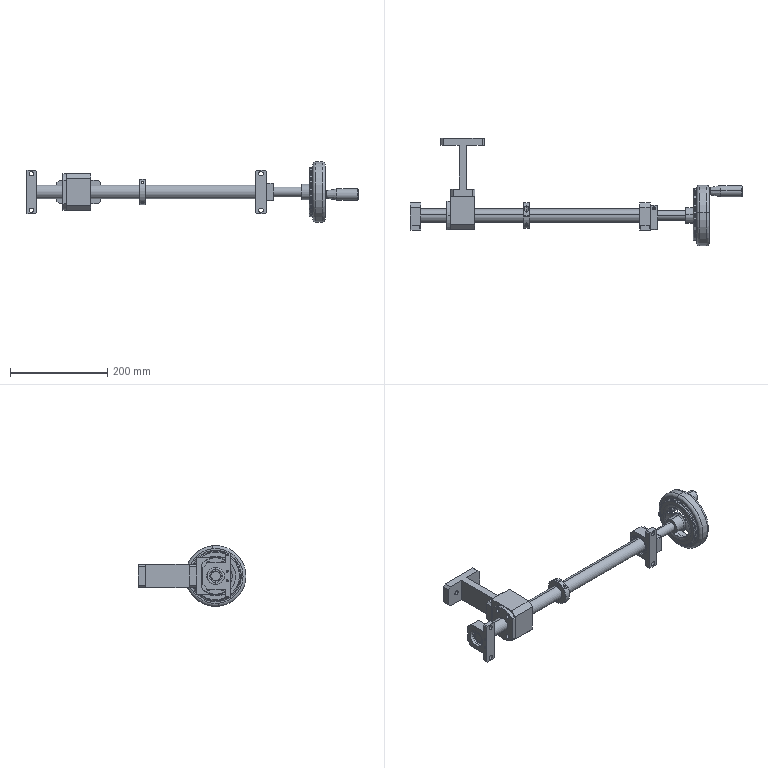Assembly | SolidWorks | mm | 14 component files | 14 solids | 512 faces | box 682.5 x 221.9 x 125 mm | volume 1080889 mm3 | cylinder 187 | plane 168 | cone 87 | torus 68 | spline 2 | commonest cylinder face diameters 9 x24 4.2 x14 42 x12 20 x11 5 x8 6.8 x8 27 x8 35 x8
Bill of materials:
GB-T276  6004RZ | 2 | '- | Short annular body with concentric outer ring and inner ring separated by a recessed annular gap; bearing-like appearance.
PHSLN_HANDLE125 | 1 |  | Axisymmetric elongated body: a cylindrical section that tapers in a cone to a shorter section, ending in a small-diameter cylindrical tip.
PHSLN125_1_1 | 1 | '- | Wheel-like disc with a thick rounded outer rim, a recessed web with two curved openings, a central hub with a keyed bore, a rear cylindrical boss, and an off-centre hole in the rim.
PHSLN125_SCREW_SCREW | 1 |  | Stepped cylindrical pin with a reduced-diameter neck between two collars, ending in a forked (clevis-like) end with a through slot and a cross hole through both prongs.
TC020.05-01 | 1 | Q235A | Rectangular block with chamfered edges, a large through bore, a narrow slit running from the bore to one end of the block, two smaller through holes at the other end, and a small hole in the top face.
TC020.05-02 | 2 | Q235A | Block with a mounting flange: a rectangular base plate with two through holes, joined to a thicker body with a large round bore that has an internal step/groove and chamfered outer corners.
TC020.05-03 | 1 | 45 Steel | Long slender stepped shaft: a main cylindrical section, a reduced section, and a small end spigot, with short end steps at the opposite end.
TC020.05-04 | 1 | Q235A | Near-square prismatic block with a large round through bore and one chamfered (cut) corner along its length.
TC020.05-05 | 1 | H68 | Flanged cylindrical bushing: a tubular body with a through bore, and a flange with two flat-cut sides and four through holes.
TC020.05-06 | 1 | Q235A | I-section shaped part: a central web joining two end plates of different widths, with chamfered corners and small holes in the end faces.
TC020.05-07 | 1 | Q235A | Half-ring (semicircular) clamp-like segment with a semicircular inner bore and two flat end lugs, each with a through hole.
TC020.05-08 | 1 | Q235A | C-shaped arc segment of a thick ring, about a half circle or slightly less, with flat end faces and small holes through the outer curved surface.
Mates:
1. concentric | TC020.05-04-1 face at (133.493, 30, 0) dir (-1, 0, 0) r 22 | TC020.05-05-1 face at (107.443, 30, 0) dir (1, 0, 0) r 22
2. coincident | TC020.05-04-1 face at (83.493, 59, 60) dir (-1, 0, 0) | TC020.05-05-1 face at (83.493, 0.05, 0) dir (1, 0, 0)
3. concentric | TC020.05-04-1 face at (83.493, 15.5, 25.115) dir (-1, 0, 0) r 3.4 | TC020.05-05-1 face at (131.493, 15.5, 25.115) dir (-1, 0, 0) r 4.5
4. coincident | TC020.05-02-3 face at (5, 30, 0) dir (1, 0, 0) | GB-T276  6004RZ-1 face at (5, 40, 0) dir (-1, 0, 0)
5. concentric | TC020.05-02-3 face at (5, 30, 0) dir (1, 0, 0) r 21 | GB-T276  6004RZ-1 face at (5, 30, 0) dir (-1, 0, 0) r 21
6. concentric | TC020.05-03-1 face at (587, 30, 0) dir (1, 0, 0) r 10 | GB-T276  6004RZ-1 face at (5, 30, 0) dir (-1, 0, 0) r 10
7. coincident | TC020.05-03-1 face at (17, 39.949, -1.006) dir (-1, 0, 0) | GB-T276  6004RZ-1 face at (17, 40, 0) dir (1, 0, 0)
8. concentric | TC020.05-03-1 face at (587, 30, 0) dir (1, 0, 0) r 14 | GB-T276  6004RZ-2 face at (489, 30, 0) dir (1, 0, 0) r 10
9. concentric | TC020.05-05-1 face at (103.493, 30, 0) dir (1, 0, 0) r 14 | TC020.05-03-1 face at (587, 30, 0) dir (1, 0, 0) r 14
10. coincident | TC020.05-03-1 face at (477, 43.929, -1.408) dir (1, 0, 0) | GB-T276  6004RZ-2 face at (477, 20, 0) dir (-1, 0, 0)
11. concentric | TC020.05-03-1 face at (587, 30, 0) dir (1, 0, 0) r 6 | PHSLN125-1/PHSLN125_1_1-1 face at (615, 30, 0) dir (-1, 0, 0) r 6
12. coincident | TC020.05-03-1 face at (567, 39.949, -1.006) dir (1, 0, 0) | PHSLN125-1/PHSLN125_1_1-1 face at (567, 30, 0) dir (-1, 0, 0)
13. concentric | TC020.05-03-1 face at (587, 30, 0) dir (1, 0, 0) r 14 | TC020.05-02-4 face at (489, 30, 0) dir (-1, 0, 0) r 21
14. coincident | GB-T276  6004RZ-2 face at (489, 12.5, 0) dir (1, 0, 0) | TC020.05-02-4 face at (489, 30, 0) dir (-1, 0, 0)
15. coincident | TC020.05-02-3 face at (22, 0, -45) dir (0, -1, 0) | TC020.05-02-4 face at (472, 0, 45) dir (0, -1, 0)
16. coincident | TC020.05-03-1 face at (561.949, 36.751, 1.328) dir (0, -0.1006, -0.9949) | PHSLN125-1/PHSLN125_1_1-1 face at (615, 37.962, 1.205) dir (0, -0.1006, -0.9949)
17. coincident | TC020.05-01-1 face at (494, 51, -17.5) dir (-1, 0, 0) | TC020.05-02-4 face at (494, 0, -45) dir (1, 0, 0)
18. concentric | TC020.05-01-1 face at (494, 6, 10) dir (1, 0, 0) r 3 | TC020.05-02-4 face at (494, 6, 10) dir (1, 0, 0) r 2.1
19. concentric | TC020.05-01-1 face at (494, 6, -10) dir (1, 0, 0) r 3 | TC020.05-02-4 face at (494, 6, -10) dir (1, 0, 0) r 2.1
20. coincident | TC020.05-04-1 face at (83.493, 69, -38) dir (0, 1, 0) | TC020.05-06-2 face at (83.493, 69, 24) dir (0, -1, 0)
21. concentric | TC020.05-04-1 face at (124.493, 69, 16) dir (0, 1, 0) r 2.5 | TC020.05-06-2 face at (124.493, 119, 16) dir (0, -1, 0) r 3.5
22. concentric | TC020.05-04-1 face at (92.493, 69, -16) dir (0, 1, 0) r 2.5 | TC020.05-06-2 face at (92.493, 119, -16) dir (0, -1, 0) r 3.5
23. parallel | TC020.05-02-3 face at (22, 56, 27.5) dir (0, 1, 0) | TC020.05-06-2 face at (153.493, 189.4, 24) dir (0, 1, 0)
24. distance | TC020.05-05-1 face at (75.493, 11.25, 0) dir (-1, 0, 0) | TC020.05-02-3 face at (22, 0, 45) dir (1, 0, 0)
25. concentric | TC020.05-03-1 face at (587, 30, 0) dir (1, 0, 0) r 14 | TC020.05-07-1 face at (239.493, 30, 0) dir (-1, 0, 0) r 14
26. concentric | TC020.05-03-1 face at (587, 30, 0) dir (1, 0, 0) r 14 | TC020.05-08-1 face at (239.493, 30, 0) dir (-1, 0, 0) r 14
27. coincident | TC020.05-07-1 face at (245.493, 43.969, 0.9288) dir (1, 0, 0) | TC020.05-08-1 face at (245.493, 16.031, -0.9288) dir (1, 0, 0)
28. parallel | TC020.05-07-1 face at (233.493, 29.273, 26.009) dir (0, -0.9978, -0.06635) | TC020.05-08-1 face at (233.493, 30.727, -26.009) dir (0, 0.9978, 0.06635)
29. distance | TC020.05-07-1 face at (233.493, 43.969, 0.9288) dir (-1, 0, 0) | TC020.05-04-1 face at (133.493, 59, 60) dir (1, 0, 0)
30. distance | PHSLN125_SCREW_SCREW-1 plane at (34.5, 50.5, 0) dir (-1, 0, 0) | PHSLN125_1_1-1 plane at (34.5, 0, 0) dir (1, 0, 0)
31. coincident | PHSLN125_1_1-1 axis at (80.9, 50.5, 0) dir (-1, 0, 0) | PHSLN125_SCREW_SCREW-1 axis at (-46.4, 50.5, 0) dir (1, 0, 0)
32. coincident | PHSLN125_1_1-1 axis at (80.9, 50.5, 0) dir (-1, 0, 0) | PHSLN125_SCREW_SCREW-1 axis at (-46.4, 50.5, 0) dir (1, 0, 0)
33. coincident | PHSLN125_1_1-1 axis at (80.9, 50.5, 0) dir (-1, 0, 0) | PHSLN125_SCREW_SCREW-1 axis at (-46.4, 50.5, 0) dir (1, 0, 0)
34. angle | PHSLN125_SCREW_SCREW-1 plane at (34.5, 50.5, 0) dir (0, 0, -1) | PHSLN125_1_1-1 plane at (0, 0, 0) dir (0, 0, -1)
35. coincident | PHSLN125_SCREW_SCREW-1 plane at (34.5, 50.5, 0) dir (-1, 0, 0) | PHSLN_HANDLE125-1 plane at (34.5, 50.5, 0) dir (1, 0, 0)
36. coincident | PHSLN125_SCREW_SCREW-1 axis at (-46.4, 50.5, 0) dir (1, 0, 0) | PHSLN_HANDLE125-1 axis at (115.4, 50.5, 0) dir (-1, 0, 0)